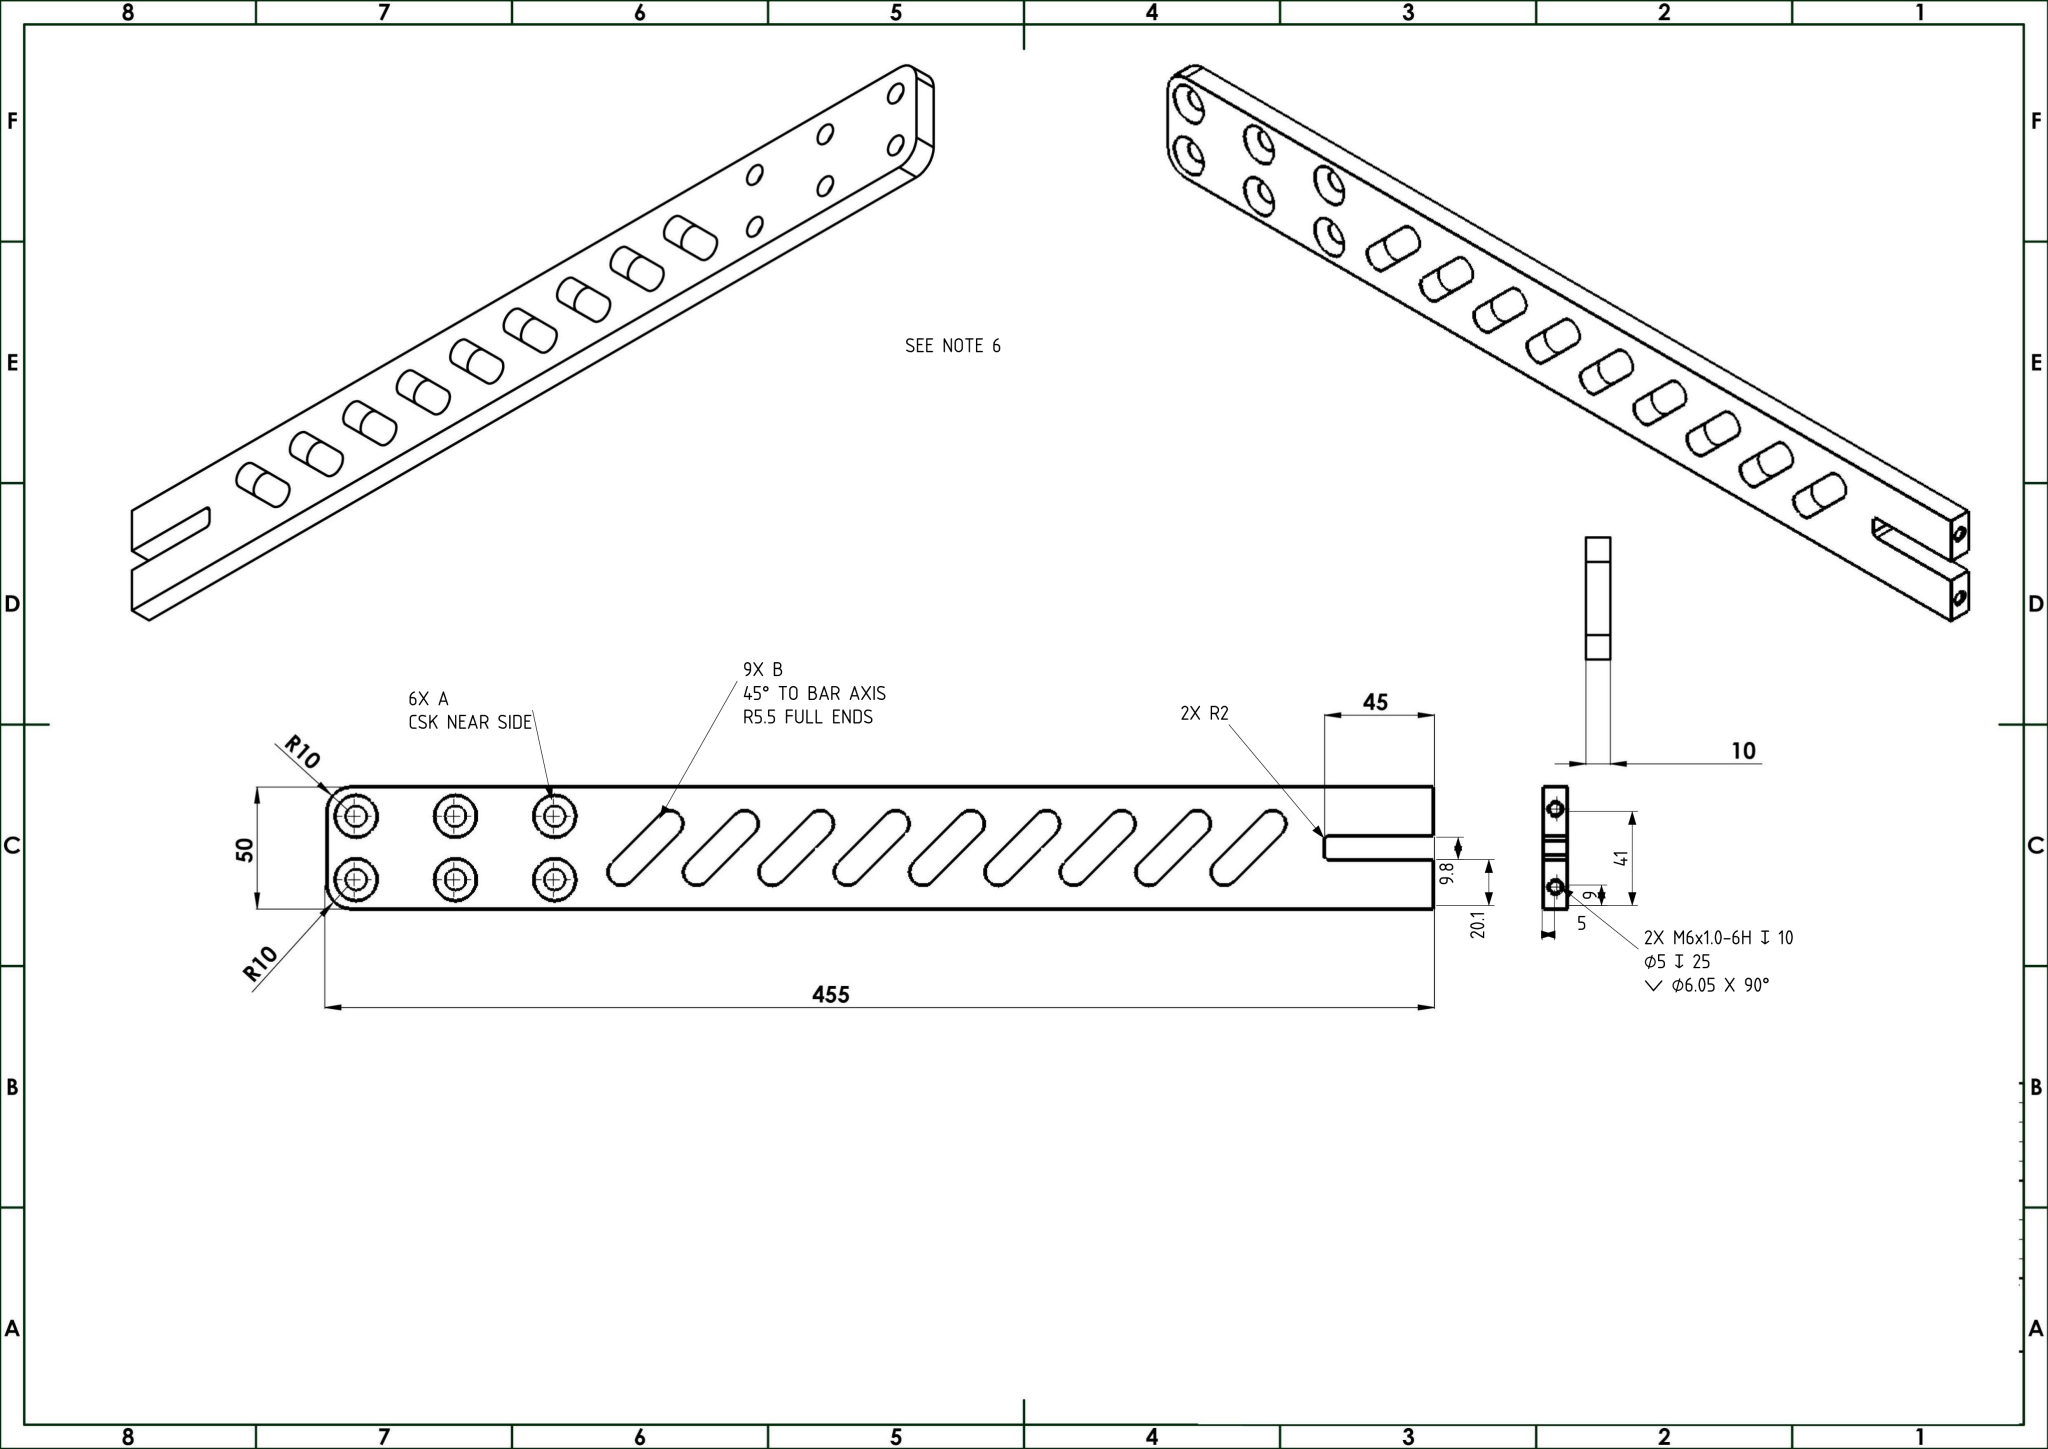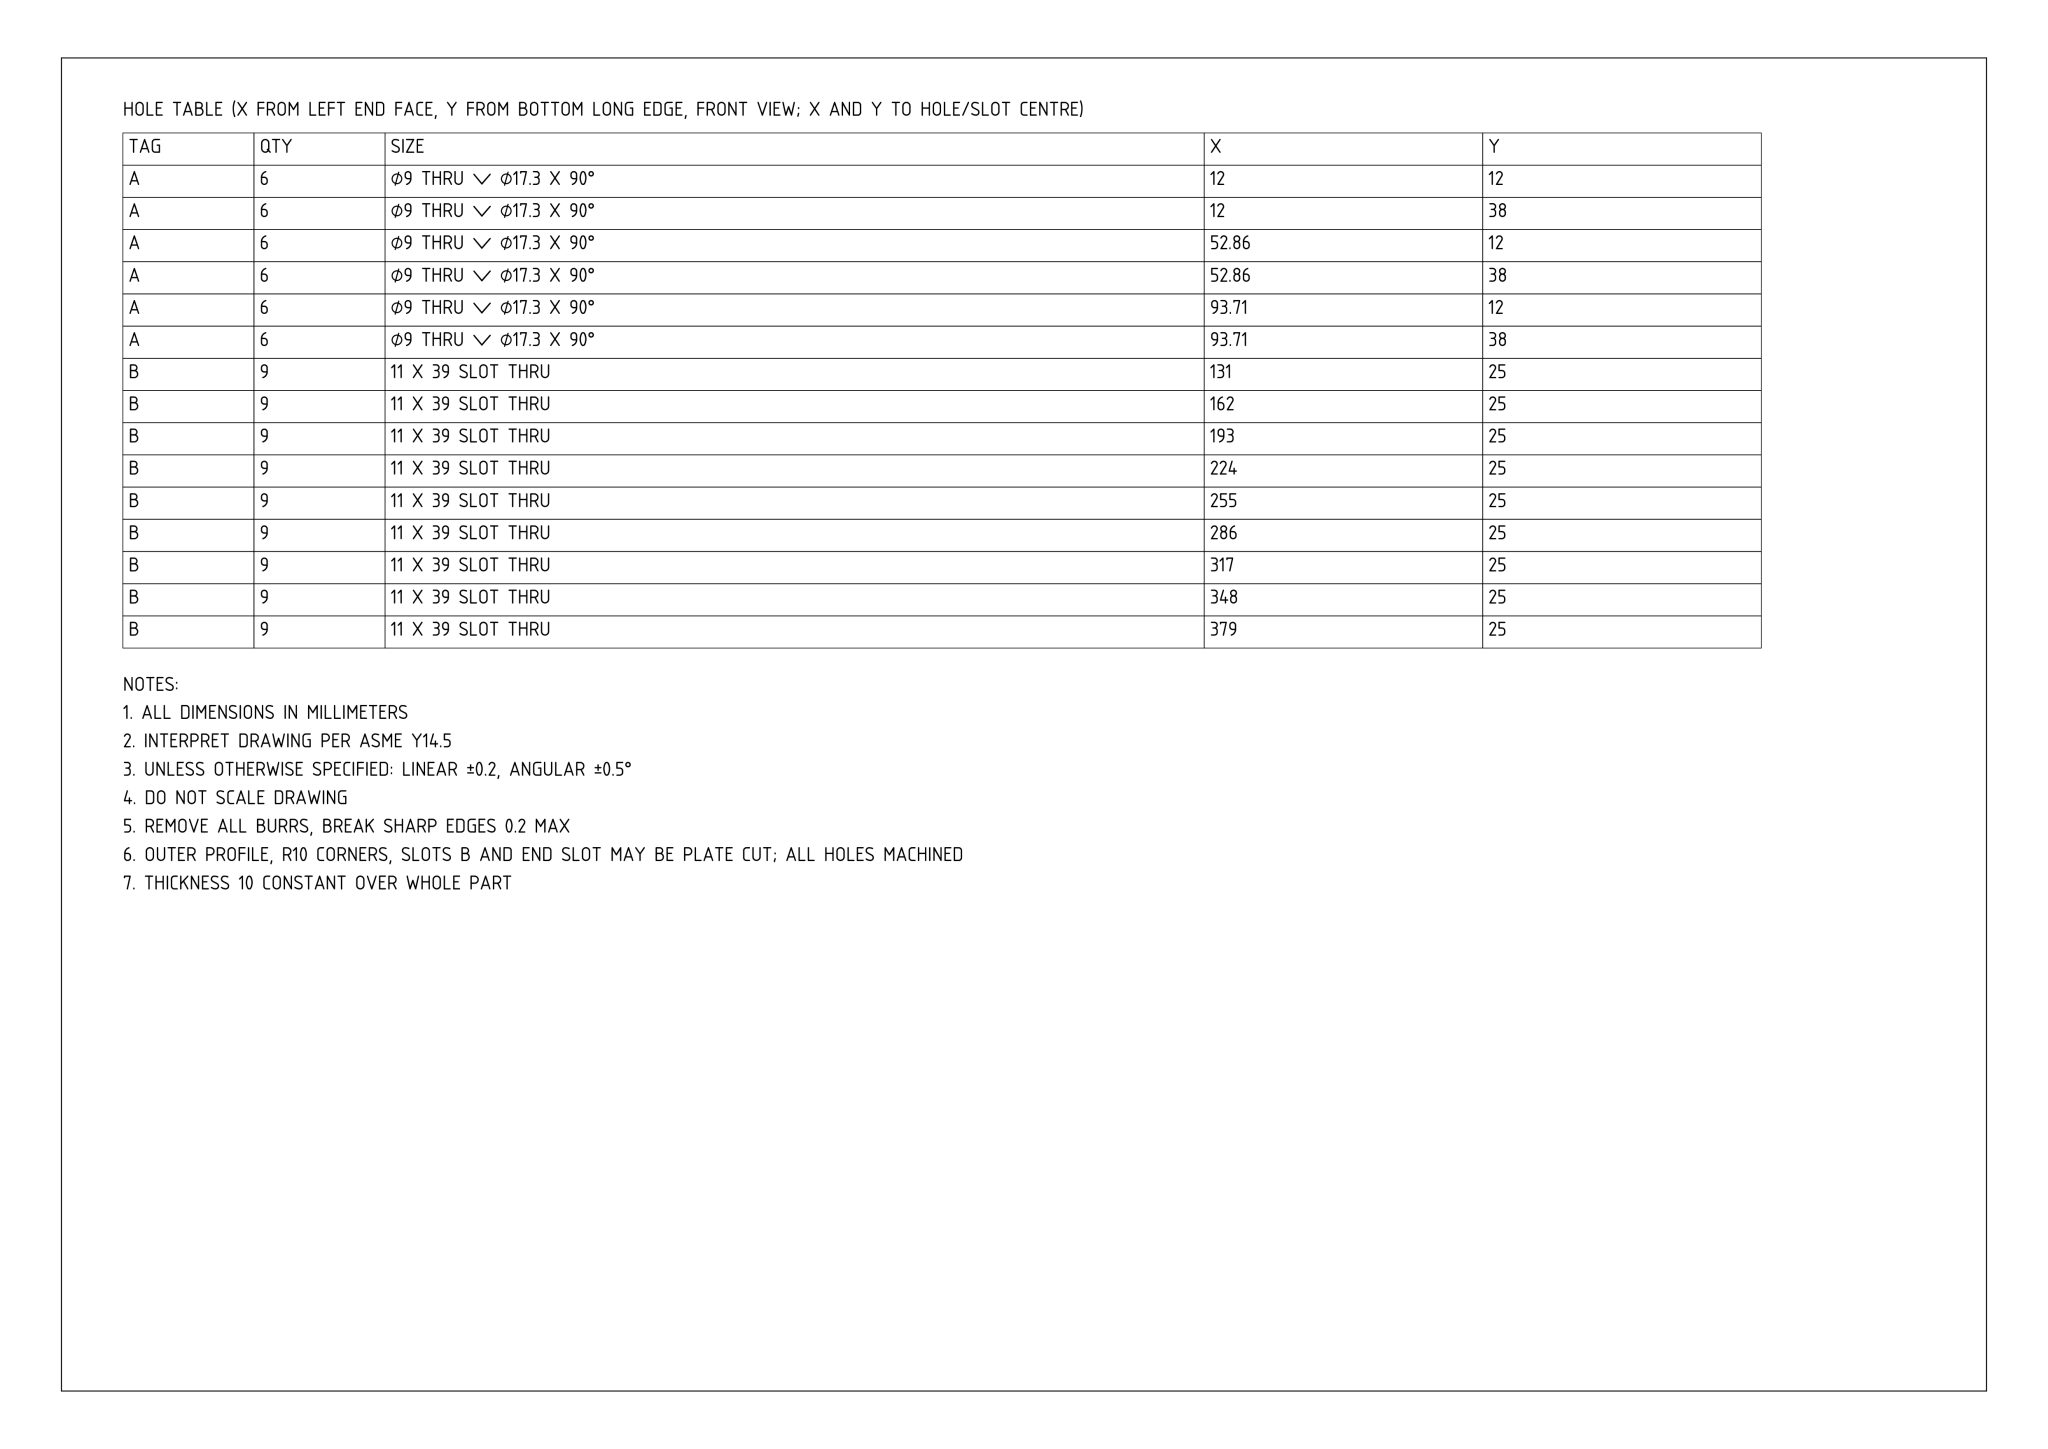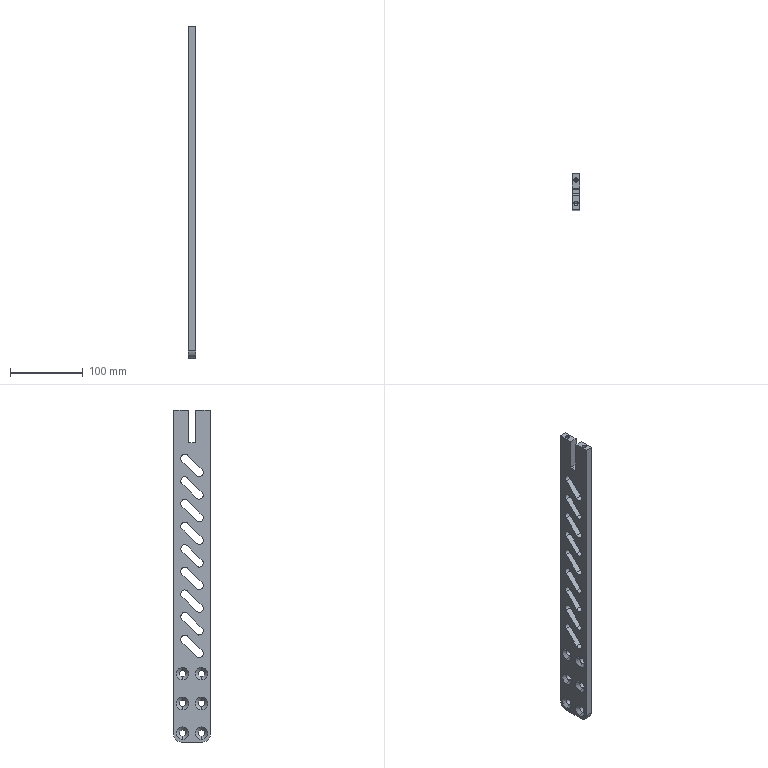Part | NX | mm | 1 solid | 95 faces | box 10 x 50 x 455 mm | volume 179672 mm3 | cylinder 47 | plane 28 | cone 20 | commonest cylinder face diameters 11 x27 9 x12 5 x4 4 x2 20 x2